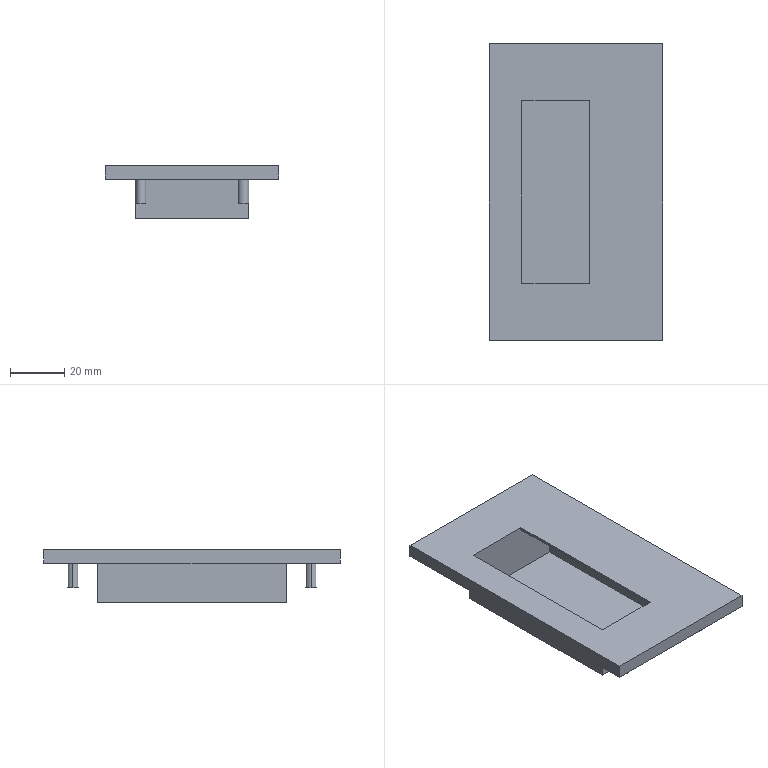Component | SolidWorks | SYM0671-81-200-1_SYMA1-51a_mis_uwuan109.5-b-1 | 1 solid | 30 faces | box 64 x 109.5 x 19.5 mm | volume 28880 mm3 | plane 22 | cylinder 8 | commonest cylinder face diameters 4 x8
build123d program:
from build123d import *

# Parameters (mm, degrees)
SKETCH_1_W           = 64
SKETCH_1_H           = 109.5
EXTRUDE1_DEPTH       = 5
SKETCH_6_W           = 42
SKETCH_6_H           = 69.5
EXTRUDE5_DEPTH       = 14.5
SKETCH1_W            = 25
SKETCH1_H            = 67.5
CUT_EXTRUDE1_DEPTH   = 18.5
SKETCH2_W            = 17.5
SKETCH2_H            = 67.5
CUT_EXTRUDE2_DEPTH   = 15
SKETCH3_R            = 2
EXTRUDE1_2_DEPTH     = 9
LPATTERN1_COUNT      = 2
LPATTERN1_PITCH      = 38
LPATTERN1_COUNT_DIR2 = 2
LPATTERN1_PITCH_DIR2 = 88


with BuildPart() as part:
    # Sketch 1 → Extrude1 (new body)
    with BuildSketch(Plane.XY):
        Rectangle(SKETCH_1_W, SKETCH_1_H)
    extrude(amount=EXTRUDE1_DEPTH)

    # Sketch 6 → Extrude5 (add)
    with BuildSketch(Plane.XY):
        Rectangle(SKETCH_6_W, SKETCH_6_H)
    extrude(amount=-EXTRUDE5_DEPTH)

    # Sketch1 → Cut-Extrude1 (cut)
    with BuildSketch(Plane.XY.offset(5)):
        with Locations((7.5, 0)):
            Rectangle(SKETCH1_W, SKETCH1_H)
    extrude(amount=-CUT_EXTRUDE1_DEPTH, mode=Mode.SUBTRACT)

    # Sketch2 → Cut-Extrude2 (cut)
    with BuildSketch(Plane(origin=(-5, 0, 0), x_dir=(0, 0, -1), z_dir=(1, 0, 0))):
        with Locations((4.75, 0)):
            Rectangle(SKETCH2_W, SKETCH2_H)
    extrude(amount=-CUT_EXTRUDE2_DEPTH, mode=Mode.SUBTRACT)

    # Sketch3 → Extrude1_2 (add)
    with BuildSketch(Plane(origin=(0, 0, 0), x_dir=(-1, 0, 0), z_dir=(0, 0, -1))):
        with Locations(Location((19, 44, 0), (0, 0, 180))):
            Circle(SKETCH3_R)
    extrude1_2 = extrude(amount=EXTRUDE1_2_DEPTH)

    # LPattern1: Extrude1_2 2 × 2
    with Locations(*[(i * LPATTERN1_PITCH, -j * LPATTERN1_PITCH_DIR2, 0) for i in range(LPATTERN1_COUNT) for j in range(LPATTERN1_COUNT_DIR2) if (i, j) != (0, 0)]):
        add(extrude1_2)


solid = part.part

# Placed as in the assembly
solid = solid.moved(Location((0.2513, -14.857, 1051.018), (0, 0, 180)))
STEP:
#1=CARTESIAN_POINT('',(-0.6594,1.147,41.024));
#2=VERTEX_POINT('',#1);
#3=CARTESIAN_POINT('',(-0.8169,1.147,41.024));
#4=VERTEX_POINT('',#3);
#5=CARTESIAN_POINT('',(-0.7381,1.147,41.024));
#6=DIRECTION('',(0.,0.,-1.));
#7=DIRECTION('',(1.,0.,0.));
#8=AXIS2_PLACEMENT_3D('',#5,#6,#7);
#9=CIRCLE('',#8,0.07874);
#10=EDGE_CURVE('',#2,#4,#9,.T.);
#11=ORIENTED_EDGE('',*,*,#10,.F.);
#12=CARTESIAN_POINT('',(-0.6594,1.147,41.379));
#13=VERTEX_POINT('',#12);
#14=CARTESIAN_POINT('',(-0.6594,1.147,41.024));
#15=DIRECTION('',(0.,0.,1.));
#16=VECTOR('',#15,39.37);
#17=LINE('',#14,#16);
#18=EDGE_CURVE('',#2,#13,#17,.T.);
#19=ORIENTED_EDGE('',*,*,#18,.T.);
#20=CARTESIAN_POINT('',(-0.8169,1.147,41.379));
#21=VERTEX_POINT('',#20);
#22=CARTESIAN_POINT('',(-0.7381,1.147,41.379));
#23=DIRECTION('',(0.,0.,-1.));
#24=DIRECTION('',(-1.,-0.,0.));
#25=AXIS2_PLACEMENT_3D('',#22,#23,#24);
#26=CIRCLE('',#25,0.07874);
#27=EDGE_CURVE('',#13,#21,#26,.T.);
#28=ORIENTED_EDGE('',*,*,#27,.T.);
#29=CARTESIAN_POINT('',(-0.8169,1.147,41.024));
#30=DIRECTION('',(0.,0.,1.));
#31=VECTOR('',#30,39.37);
#32=LINE('',#29,#31);
#33=EDGE_CURVE('',#4,#21,#32,.T.);
#34=ORIENTED_EDGE('',*,*,#33,.F.);
#35=EDGE_LOOP('',(#11,#19,#28,#34));
#36=FACE_OUTER_BOUND('',#35,.T.);
#37=CARTESIAN_POINT('',(-0.7381,1.147,41.024));
#38=DIRECTION('',(0.,0.,1.));
#39=DIRECTION('',(-1.,0.,0.));
#40=AXIS2_PLACEMENT_3D('',#37,#38,#39);
#41=CYLINDRICAL_SURFACE('',#40,0.07874);
#42=ADVANCED_FACE('',(#36),#41,.T.);
#43=CARTESIAN_POINT('',(0.8367,1.147,41.024));
#44=VERTEX_POINT('',#43);
#45=CARTESIAN_POINT('',(0.6792,1.147,41.024));
#46=VERTEX_POINT('',#45);
#47=CARTESIAN_POINT('',(0.7579,1.147,41.024));
#48=DIRECTION('',(0.,0.,-1.));
#49=DIRECTION('',(1.,0.,0.));
#50=AXIS2_PLACEMENT_3D('',#47,#48,#49);
#51=CIRCLE('',#50,0.07874);
#52=EDGE_CURVE('',#44,#46,#51,.T.);
#53=ORIENTED_EDGE('',*,*,#52,.F.);
#54=CARTESIAN_POINT('',(0.8367,1.147,41.379));
#55=VERTEX_POINT('',#54);
#56=CARTESIAN_POINT('',(0.8367,1.147,41.024));
#57=DIRECTION('',(0.,0.,1.));
#58=VECTOR('',#57,39.37);
#59=LINE('',#56,#58);
#60=EDGE_CURVE('',#44,#55,#59,.T.);
#61=ORIENTED_EDGE('',*,*,#60,.T.);
#62=CARTESIAN_POINT('',(0.6792,1.147,41.379));
#63=VERTEX_POINT('',#62);
#64=CARTESIAN_POINT('',(0.7579,1.147,41.379));
#65=DIRECTION('',(0.,0.,-1.));
#66=DIRECTION('',(-1.,-0.,0.));
#67=AXIS2_PLACEMENT_3D('',#64,#65,#66);
#68=CIRCLE('',#67,0.07874);
#69=EDGE_CURVE('',#55,#63,#68,.T.);
#70=ORIENTED_EDGE('',*,*,#69,.T.);
#71=CARTESIAN_POINT('',(0.6792,1.147,41.024));
#72=DIRECTION('',(0.,0.,1.));
#73=VECTOR('',#72,39.37);
#74=LINE('',#71,#73);
#75=EDGE_CURVE('',#46,#63,#74,.T.);
#76=ORIENTED_EDGE('',*,*,#75,.F.);
#77=EDGE_LOOP('',(#53,#61,#70,#76));
#78=FACE_OUTER_BOUND('',#77,.T.);
#79=CARTESIAN_POINT('',(0.7579,1.147,41.024));
#80=DIRECTION('',(0.,0.,1.));
#81=DIRECTION('',(-1.,0.,0.));
#82=AXIS2_PLACEMENT_3D('',#79,#80,#81);
#83=CYLINDRICAL_SURFACE('',#82,0.07874);
#84=ADVANCED_FACE('',(#78),#83,.T.);
#85=CARTESIAN_POINT('',(-0.6594,-2.317,41.024));
#86=VERTEX_POINT('',#85);
#87=CARTESIAN_POINT('',(-0.8169,-2.317,41.024));
#88=VERTEX_POINT('',#87);
#89=CARTESIAN_POINT('',(-0.7381,-2.317,41.024));
#90=DIRECTION('',(0.,0.,-1.));
#91=DIRECTION('',(1.,0.,0.));
#92=AXIS2_PLACEMENT_3D('',#89,#90,#91);
#93=CIRCLE('',#92,0.07874);
#94=EDGE_CURVE('',#86,#88,#93,.T.);
#95=ORIENTED_EDGE('',*,*,#94,.F.);
#96=CARTESIAN_POINT('',(-0.6594,-2.317,41.379));
#97=VERTEX_POINT('',#96);
#98=CARTESIAN_POINT('',(-0.6594,-2.317,41.024));
#99=DIRECTION('',(0.,0.,1.));
#100=VECTOR('',#99,39.37);
#101=LINE('',#98,#100);
#102=EDGE_CURVE('',#86,#97,#101,.T.);
#103=ORIENTED_EDGE('',*,*,#102,.T.);
#104=CARTESIAN_POINT('',(-0.8169,-2.317,41.379));
#105=VERTEX_POINT('',#104);
#106=CARTESIAN_POINT('',(-0.7381,-2.317,41.379));
#107=DIRECTION('',(0.,0.,-1.));
#108=DIRECTION('',(-1.,0.,0.));
#109=AXIS2_PLACEMENT_3D('',#106,#107,#108);
#110=CIRCLE('',#109,0.07874);
#111=EDGE_CURVE('',#97,#105,#110,.T.);
#112=ORIENTED_EDGE('',*,*,#111,.T.);
#113=CARTESIAN_POINT('',(-0.8169,-2.317,41.024));
#114=DIRECTION('',(0.,0.,1.));
#115=VECTOR('',#114,39.37);
#116=LINE('',#113,#115);
#117=EDGE_CURVE('',#88,#105,#116,.T.);
#118=ORIENTED_EDGE('',*,*,#117,.F.);
#119=EDGE_LOOP('',(#95,#103,#112,#118));
#120=FACE_OUTER_BOUND('',#119,.T.);
#121=CARTESIAN_POINT('',(-0.7381,-2.317,41.024));
#122=DIRECTION('',(0.,0.,1.));
#123=DIRECTION('',(-1.,0.,0.));
#124=AXIS2_PLACEMENT_3D('',#121,#122,#123);
#125=CYLINDRICAL_SURFACE('',#124,0.07874);
#126=ADVANCED_FACE('',(#120),#125,.T.);
#127=CARTESIAN_POINT('',(0.8367,-2.317,41.024));
#128=VERTEX_POINT('',#127);
#129=CARTESIAN_POINT('',(0.6792,-2.317,41.024));
#130=VERTEX_POINT('',#129);
#131=CARTESIAN_POINT('',(0.7579,-2.317,41.024));
#132=DIRECTION('',(0.,0.,-1.));
#133=DIRECTION('',(1.,0.,0.));
#134=AXIS2_PLACEMENT_3D('',#131,#132,#133);
#135=CIRCLE('',#134,0.07874);
#136=EDGE_CURVE('',#128,#130,#135,.T.);
#137=ORIENTED_EDGE('',*,*,#136,.F.);
#138=CARTESIAN_POINT('',(0.8367,-2.317,41.379));
#139=VERTEX_POINT('',#138);
#140=CARTESIAN_POINT('',(0.8367,-2.317,41.024));
#141=DIRECTION('',(0.,0.,1.));
#142=VECTOR('',#141,39.37);
#143=LINE('',#140,#142);
#144=EDGE_CURVE('',#128,#139,#143,.T.);
#145=ORIENTED_EDGE('',*,*,#144,.T.);
#146=CARTESIAN_POINT('',(0.6792,-2.317,41.379));
#147=VERTEX_POINT('',#146);
#148=CARTESIAN_POINT('',(0.7579,-2.317,41.379));
#149=DIRECTION('',(0.,0.,-1.));
#150=DIRECTION('',(-1.,0.,0.));
#151=AXIS2_PLACEMENT_3D('',#148,#149,#150);
#152=CIRCLE('',#151,0.07874);
#153=EDGE_CURVE('',#139,#147,#152,.T.);
#154=ORIENTED_EDGE('',*,*,#153,.T.);
#155=CARTESIAN_POINT('',(0.6792,-2.317,41.024));
#156=DIRECTION('',(0.,0.,1.));
#157=VECTOR('',#156,39.37);
#158=LINE('',#155,#157);
#159=EDGE_CURVE('',#130,#147,#158,.T.);
#160=ORIENTED_EDGE('',*,*,#159,.F.);
#161=EDGE_LOOP('',(#137,#145,#154,#160));
#162=FACE_OUTER_BOUND('',#161,.T.);
#163=CARTESIAN_POINT('',(0.7579,-2.317,41.024));
#164=DIRECTION('',(0.,0.,1.));
#165=DIRECTION('',(-1.,0.,0.));
#166=AXIS2_PLACEMENT_3D('',#163,#164,#165);
#167=CYLINDRICAL_SURFACE('',#166,0.07874);
#168=ADVANCED_FACE('',(#162),#167,.T.);
#169=CARTESIAN_POINT('',(0.7579,-2.317,41.379));
#170=DIRECTION('',(0.,0.,-1.));
#171=DIRECTION('',(-1.,0.,0.));
#172=AXIS2_PLACEMENT_3D('',#169,#170,#171);
#173=CIRCLE('',#172,0.07874);
#174=EDGE_CURVE('',#147,#139,#173,.T.);
#175=ORIENTED_EDGE('',*,*,#174,.F.);
#176=ORIENTED_EDGE('',*,*,#153,.F.);
#177=EDGE_LOOP('',(#175,#176));
#178=FACE_BOUND('',#177,.T.);
#179=CARTESIAN_POINT('',(0.8367,0.7832,41.379));
#180=VERTEX_POINT('',#179);
#181=CARTESIAN_POINT('',(-0.8169,0.7832,41.379));
#182=VERTEX_POINT('',#181);
#183=CARTESIAN_POINT('',(-0.8169,0.7832,41.379));
#184=DIRECTION('',(-1.,-0.,0.));
#185=VECTOR('',#184,39.37);
#186=LINE('',#183,#185);
#187=EDGE_CURVE('',#180,#182,#186,.T.);
#188=ORIENTED_EDGE('',*,*,#187,.T.);
#189=CARTESIAN_POINT('',(-0.8169,-1.953,41.379));
#190=VERTEX_POINT('',#189);
#191=CARTESIAN_POINT('',(-0.8169,-1.953,41.379));
#192=DIRECTION('',(0.,-1.,0.));
#193=VECTOR('',#192,39.37);
#194=LINE('',#191,#193);
#195=EDGE_CURVE('',#182,#190,#194,.T.);
#196=ORIENTED_EDGE('',*,*,#195,.T.);
#197=CARTESIAN_POINT('',(0.8367,-1.953,41.379));
#198=VERTEX_POINT('',#197);
#199=CARTESIAN_POINT('',(-0.8169,-1.953,41.379));
#200=DIRECTION('',(1.,0.,0.));
#201=VECTOR('',#200,39.37);
#202=LINE('',#199,#201);
#203=EDGE_CURVE('',#190,#198,#202,.T.);
#204=ORIENTED_EDGE('',*,*,#203,.T.);
#205=CARTESIAN_POINT('',(0.8367,-1.953,41.379));
#206=DIRECTION('',(-0.,1.,0.));
#207=VECTOR('',#206,39.37);
#208=LINE('',#205,#207);
#209=EDGE_CURVE('',#198,#180,#208,.T.);
#210=ORIENTED_EDGE('',*,*,#209,.T.);
#211=EDGE_LOOP('',(#188,#196,#204,#210));
#212=FACE_BOUND('',#211,.T.);
#213=CARTESIAN_POINT('',(1.27,-2.74,41.379));
#214=VERTEX_POINT('',#213);
#215=CARTESIAN_POINT('',(1.27,1.571,41.379));
#216=VERTEX_POINT('',#215);
#217=CARTESIAN_POINT('',(1.27,-2.74,41.379));
#218=DIRECTION('',(-0.,1.,0.));
#219=VECTOR('',#218,39.37);
#220=LINE('',#217,#219);
#221=EDGE_CURVE('',#214,#216,#220,.T.);
#222=ORIENTED_EDGE('',*,*,#221,.F.);
#223=CARTESIAN_POINT('',(-1.25,-2.74,41.379));
#224=VERTEX_POINT('',#223);
#225=CARTESIAN_POINT('',(1.27,-2.74,41.379));
#226=DIRECTION('',(1.,0.,0.));
#227=VECTOR('',#226,39.37);
#228=LINE('',#225,#227);
#229=EDGE_CURVE('',#224,#214,#228,.T.);
#230=ORIENTED_EDGE('',*,*,#229,.F.);
#231=CARTESIAN_POINT('',(-1.25,1.571,41.379));
#232=VERTEX_POINT('',#231);
#233=CARTESIAN_POINT('',(-1.25,-2.74,41.379));
#234=DIRECTION('',(0.,-1.,0.));
#235=VECTOR('',#234,39.37);
#236=LINE('',#233,#235);
#237=EDGE_CURVE('',#232,#224,#236,.T.);
#238=ORIENTED_EDGE('',*,*,#237,.F.);
#239=CARTESIAN_POINT('',(1.27,1.571,41.379));
#240=DIRECTION('',(-1.,-0.,0.));
#241=VECTOR('',#240,39.37);
#242=LINE('',#239,#241);
#243=EDGE_CURVE('',#216,#232,#242,.T.);
#244=ORIENTED_EDGE('',*,*,#243,.F.);
#245=EDGE_LOOP('',(#222,#230,#238,#244));
#246=FACE_OUTER_BOUND('',#245,.T.);
#247=CARTESIAN_POINT('',(-0.7381,-2.317,41.379));
#248=DIRECTION('',(0.,0.,-1.));
#249=DIRECTION('',(-1.,0.,0.));
#250=AXIS2_PLACEMENT_3D('',#247,#248,#249);
#251=CIRCLE('',#250,0.07874);
#252=EDGE_CURVE('',#105,#97,#251,.T.);
#253=ORIENTED_EDGE('',*,*,#252,.F.);
#254=ORIENTED_EDGE('',*,*,#111,.F.);
#255=EDGE_LOOP('',(#253,#254));
#256=FACE_BOUND('',#255,.T.);
#257=CARTESIAN_POINT('',(0.7579,1.147,41.379));
#258=DIRECTION('',(0.,0.,-1.));
#259=DIRECTION('',(-1.,0.,0.));
#260=AXIS2_PLACEMENT_3D('',#257,#258,#259);
#261=CIRCLE('',#260,0.07874);
#262=EDGE_CURVE('',#63,#55,#261,.T.);
#263=ORIENTED_EDGE('',*,*,#262,.F.);
#264=ORIENTED_EDGE('',*,*,#69,.F.);
#265=EDGE_LOOP('',(#263,#264));
#266=FACE_BOUND('',#265,.T.);
#267=CARTESIAN_POINT('',(-0.7381,1.147,41.379));
#268=DIRECTION('',(0.,0.,-1.));
#269=DIRECTION('',(-1.,0.,0.));
#270=AXIS2_PLACEMENT_3D('',#267,#268,#269);
#271=CIRCLE('',#270,0.07874);
#272=EDGE_CURVE('',#21,#13,#271,.T.);
#273=ORIENTED_EDGE('',*,*,#272,.F.);
#274=ORIENTED_EDGE('',*,*,#27,.F.);
#275=EDGE_LOOP('',(#273,#274));
#276=FACE_BOUND('',#275,.T.);
#277=CARTESIAN_POINT('',(1.27,1.571,41.379));
#278=DIRECTION('',(0.,0.,1.));
#279=DIRECTION('',(-1.,-0.,0.));
#280=AXIS2_PLACEMENT_3D('',#277,#278,#279);
#281=PLANE('',#280);
#282=ADVANCED_FACE('',(#178,#212,#246,#256,#266,#276),#281,.F.);
#283=ORIENTED_EDGE('',*,*,#221,.T.);
#284=CARTESIAN_POINT('',(1.27,1.571,41.575));
#285=VERTEX_POINT('',#284);
#286=CARTESIAN_POINT('',(1.27,1.571,41.575));
#287=DIRECTION('',(0.,0.,-1.));
#288=VECTOR('',#287,39.37);
#289=LINE('',#286,#288);
#290=EDGE_CURVE('',#285,#216,#289,.T.);
#291=ORIENTED_EDGE('',*,*,#290,.F.);
#292=CARTESIAN_POINT('',(1.27,-2.74,41.575));
#293=VERTEX_POINT('',#292);
#294=CARTESIAN_POINT('',(1.27,-2.74,41.575));
#295=DIRECTION('',(-0.,1.,0.));
#296=VECTOR('',#295,39.37);
#297=LINE('',#294,#296);
#298=EDGE_CURVE('',#293,#285,#297,.T.);
#299=ORIENTED_EDGE('',*,*,#298,.F.);
#300=CARTESIAN_POINT('',(1.27,-2.74,41.575));
#301=DIRECTION('',(0.,0.,-1.));
#302=VECTOR('',#301,39.37);
#303=LINE('',#300,#302);
#304=EDGE_CURVE('',#293,#214,#303,.T.);
#305=ORIENTED_EDGE('',*,*,#304,.T.);
#306=EDGE_LOOP('',(#283,#291,#299,#305));
#307=FACE_OUTER_BOUND('',#306,.T.);
#308=CARTESIAN_POINT('',(1.27,-2.74,41.575));
#309=DIRECTION('',(-1.,-0.,0.));
#310=DIRECTION('',(0.,-1.,0.));
#311=AXIS2_PLACEMENT_3D('',#308,#309,#310);
#312=PLANE('',#311);
#313=ADVANCED_FACE('',(#307),#312,.F.);
#314=ORIENTED_EDGE('',*,*,#243,.T.);
#315=CARTESIAN_POINT('',(-1.25,1.571,41.575));
#316=VERTEX_POINT('',#315);
#317=CARTESIAN_POINT('',(-1.25,1.571,41.575));
#318=DIRECTION('',(0.,0.,-1.));
#319=VECTOR('',#318,39.37);
#320=LINE('',#317,#319);
#321=EDGE_CURVE('',#316,#232,#320,.T.);
#322=ORIENTED_EDGE('',*,*,#321,.F.);
#323=CARTESIAN_POINT('',(1.27,1.571,41.575));
#324=DIRECTION('',(-1.,-0.,0.));
#325=VECTOR('',#324,39.37);
#326=LINE('',#323,#325);
#327=EDGE_CURVE('',#285,#316,#326,.T.);
#328=ORIENTED_EDGE('',*,*,#327,.F.);
#329=ORIENTED_EDGE('',*,*,#290,.T.);
#330=EDGE_LOOP('',(#314,#322,#328,#329));
#331=FACE_OUTER_BOUND('',#330,.T.);
#332=CARTESIAN_POINT('',(1.27,1.571,41.575));
#333=DIRECTION('',(0.,-1.,0.));
#334=DIRECTION('',(1.,0.,0.));
#335=AXIS2_PLACEMENT_3D('',#332,#333,#334);
#336=PLANE('',#335);
#337=ADVANCED_FACE('',(#331),#336,.F.);
#338=ORIENTED_EDGE('',*,*,#237,.T.);
#339=CARTESIAN_POINT('',(-1.25,-2.74,41.575));
#340=VERTEX_POINT('',#339);
#341=CARTESIAN_POINT('',(-1.25,-2.74,41.575));
#342=DIRECTION('',(0.,0.,-1.));
#343=VECTOR('',#342,39.37);
#344=LINE('',#341,#343);
#345=EDGE_CURVE('',#340,#224,#344,.T.);
#346=ORIENTED_EDGE('',*,*,#345,.F.);
#347=CARTESIAN_POINT('',(-1.25,-2.74,41.575));
#348=DIRECTION('',(0.,-1.,0.));
#349=VECTOR('',#348,39.37);
#350=LINE('',#347,#349);
#351=EDGE_CURVE('',#316,#340,#350,.T.);
#352=ORIENTED_EDGE('',*,*,#351,.F.);
#353=ORIENTED_EDGE('',*,*,#321,.T.);
#354=EDGE_LOOP('',(#338,#346,#352,#353));
#355=FACE_OUTER_BOUND('',#354,.T.);
#356=CARTESIAN_POINT('',(-1.25,-2.74,41.575));
#357=DIRECTION('',(1.,0.,0.));
#358=DIRECTION('',(-0.,1.,0.));
#359=AXIS2_PLACEMENT_3D('',#356,#357,#358);
#360=PLANE('',#359);
#361=ADVANCED_FACE('',(#355),#360,.F.);
#362=ORIENTED_EDGE('',*,*,#229,.T.);
#363=ORIENTED_EDGE('',*,*,#304,.F.);
#364=CARTESIAN_POINT('',(1.27,-2.74,41.575));
#365=DIRECTION('',(1.,0.,0.));
#366=VECTOR('',#365,39.37);
#367=LINE('',#364,#366);
#368=EDGE_CURVE('',#340,#293,#367,.T.);
#369=ORIENTED_EDGE('',*,*,#368,.F.);
#370=ORIENTED_EDGE('',*,*,#345,.T.);
#371=EDGE_LOOP('',(#362,#363,#369,#370));
#372=FACE_OUTER_BOUND('',#371,.T.);
#373=CARTESIAN_POINT('',(1.27,-2.74,41.575));
#374=DIRECTION('',(-0.,1.,0.));
#375=DIRECTION('',(-1.,-0.,0.));
#376=AXIS2_PLACEMENT_3D('',#373,#374,#375);
#377=PLANE('',#376);
#378=ADVANCED_FACE('',(#372),#377,.F.);
#379=CARTESIAN_POINT('',(0.2067,0.7438,41.575));
#380=VERTEX_POINT('',#379);
#381=CARTESIAN_POINT('',(-0.7775,0.7438,41.575));
#382=VERTEX_POINT('',#381);
#383=CARTESIAN_POINT('',(0.2067,0.7438,41.575));
#384=DIRECTION('',(-1.,-0.,0.));
#385=VECTOR('',#384,39.37);
#386=LINE('',#383,#385);
#387=EDGE_CURVE('',#380,#382,#386,.T.);
#388=ORIENTED_EDGE('',*,*,#387,.F.);
#389=CARTESIAN_POINT('',(0.2067,-1.914,41.575));
#390=VERTEX_POINT('',#389);
#391=CARTESIAN_POINT('',(0.2067,-1.914,41.575));
#392=DIRECTION('',(-0.,1.,0.));
#393=VECTOR('',#392,39.37);
#394=LINE('',#391,#393);
#395=EDGE_CURVE('',#390,#380,#394,.T.);
#396=ORIENTED_EDGE('',*,*,#395,.F.);
#397=CARTESIAN_POINT('',(-0.7775,-1.914,41.575));
#398=VERTEX_POINT('',#397);
#399=CARTESIAN_POINT('',(-0.7775,-1.914,41.575));
#400=DIRECTION('',(1.,0.,0.));
#401=VECTOR('',#400,39.37);
#402=LINE('',#399,#401);
#403=EDGE_CURVE('',#398,#390,#402,.T.);
#404=ORIENTED_EDGE('',*,*,#403,.F.);
#405=CARTESIAN_POINT('',(-0.7775,0.7438,41.575));
#406=DIRECTION('',(0.,-1.,0.));
#407=VECTOR('',#406,39.37);
#408=LINE('',#405,#407);
#409=EDGE_CURVE('',#382,#398,#408,.T.);
#410=ORIENTED_EDGE('',*,*,#409,.F.);
#411=EDGE_LOOP('',(#388,#396,#404,#410));
#412=FACE_BOUND('',#411,.T.);
#413=ORIENTED_EDGE('',*,*,#298,.T.);
#414=ORIENTED_EDGE('',*,*,#327,.T.);
#415=ORIENTED_EDGE('',*,*,#351,.T.);
#416=ORIENTED_EDGE('',*,*,#368,.T.);
#417=EDGE_LOOP('',(#413,#414,#415,#416));
#418=FACE_OUTER_BOUND('',#417,.T.);
#419=CARTESIAN_POINT('',(1.27,1.571,41.575));
#420=DIRECTION('',(0.,0.,1.));
#421=DIRECTION('',(-1.,-0.,0.));
#422=AXIS2_PLACEMENT_3D('',#419,#420,#421);
#423=PLANE('',#422);
#424=ADVANCED_FACE('',(#412,#418),#423,.T.);
#425=ORIENTED_EDGE('',*,*,#195,.F.);
#426=CARTESIAN_POINT('',(-0.8169,0.7832,40.808));
#427=VERTEX_POINT('',#426);
#428=CARTESIAN_POINT('',(-0.8169,0.7832,40.808));
#429=DIRECTION('',(0.,0.,1.));
#430=VECTOR('',#429,39.37);
#431=LINE('',#428,#430);
#432=EDGE_CURVE('',#427,#182,#431,.T.);
#433=ORIENTED_EDGE('',*,*,#432,.F.);
#434=CARTESIAN_POINT('',(-0.8169,-1.953,40.808));
#435=VERTEX_POINT('',#434);
#436=CARTESIAN_POINT('',(-0.8169,-1.953,40.808));
#437=DIRECTION('',(0.,-1.,0.));
#438=VECTOR('',#437,39.37);
#439=LINE('',#436,#438);
#440=EDGE_CURVE('',#427,#435,#439,.T.);
#441=ORIENTED_EDGE('',*,*,#440,.T.);
#442=CARTESIAN_POINT('',(-0.8169,-1.953,40.808));
#443=DIRECTION('',(0.,0.,1.));
#444=VECTOR('',#443,39.37);
#445=LINE('',#442,#444);
#446=EDGE_CURVE('',#435,#190,#445,.T.);
#447=ORIENTED_EDGE('',*,*,#446,.T.);
#448=EDGE_LOOP('',(#425,#433,#441,#447));
#449=FACE_OUTER_BOUND('',#448,.T.);
#450=CARTESIAN_POINT('',(-0.8169,-1.953,40.808));
#451=DIRECTION('',(-1.,-0.,0.));
#452=DIRECTION('',(0.,-1.,0.));
#453=AXIS2_PLACEMENT_3D('',#450,#451,#452);
#454=PLANE('',#453);
#455=ADVANCED_FACE('',(#449),#454,.T.);
#456=ORIENTED_EDGE('',*,*,#187,.F.);
#457=CARTESIAN_POINT('',(0.8367,0.7832,40.808));
#458=VERTEX_POINT('',#457);
#459=CARTESIAN_POINT('',(0.8367,0.7832,40.808));
#460=DIRECTION('',(0.,0.,1.));
#461=VECTOR('',#460,39.37);
#462=LINE('',#459,#461);
#463=EDGE_CURVE('',#458,#180,#462,.T.);
#464=ORIENTED_EDGE('',*,*,#463,.F.);
#465=CARTESIAN_POINT('',(-0.8169,0.7832,40.808));
#466=DIRECTION('',(-1.,-0.,0.));
#467=VECTOR('',#466,39.37);
#468=LINE('',#465,#467);
#469=EDGE_CURVE('',#458,#427,#468,.T.);
#470=ORIENTED_EDGE('',*,*,#469,.T.);
#471=ORIENTED_EDGE('',*,*,#432,.T.);
#472=EDGE_LOOP('',(#456,#464,#470,#471));
#473=FACE_OUTER_BOUND('',#472,.T.);
#474=CARTESIAN_POINT('',(-0.8169,0.7832,40.808));
#475=DIRECTION('',(-0.,1.,0.));
#476=DIRECTION('',(-1.,-0.,0.));
#477=AXIS2_PLACEMENT_3D('',#474,#475,#476);
#478=PLANE('',#477);
#479=ADVANCED_FACE('',(#473),#478,.T.);
#480=ORIENTED_EDGE('',*,*,#209,.F.);
#481=CARTESIAN_POINT('',(0.8367,-1.953,40.808));
#482=VERTEX_POINT('',#481);
#483=CARTESIAN_POINT('',(0.8367,-1.953,40.808));
#484=DIRECTION('',(0.,0.,1.));
#485=VECTOR('',#484,39.37);
#486=LINE('',#483,#485);
#487=EDGE_CURVE('',#482,#198,#486,.T.);
#488=ORIENTED_EDGE('',*,*,#487,.F.);
#489=CARTESIAN_POINT('',(0.8367,-1.953,40.808));
#490=DIRECTION('',(-0.,1.,0.));
#491=VECTOR('',#490,39.37);
#492=LINE('',#489,#491);
#493=EDGE_CURVE('',#482,#458,#492,.T.);
#494=ORIENTED_EDGE('',*,*,#493,.T.);
#495=ORIENTED_EDGE('',*,*,#463,.T.);
#496=EDGE_LOOP('',(#480,#488,#494,#495));
#497=FACE_OUTER_BOUND('',#496,.T.);
#498=CARTESIAN_POINT('',(0.8367,-1.953,40.808));
#499=DIRECTION('',(1.,0.,0.));
#500=DIRECTION('',(-0.,1.,0.));
#501=AXIS2_PLACEMENT_3D('',#498,#499,#500);
#502=PLANE('',#501);
#503=ADVANCED_FACE('',(#497),#502,.T.);
#504=ORIENTED_EDGE('',*,*,#203,.F.);
#505=ORIENTED_EDGE('',*,*,#446,.F.);
#506=CARTESIAN_POINT('',(-0.8169,-1.953,40.808));
#507=DIRECTION('',(1.,0.,0.));
#508=VECTOR('',#507,39.37);
#509=LINE('',#506,#508);
#510=EDGE_CURVE('',#435,#482,#509,.T.);
#511=ORIENTED_EDGE('',*,*,#510,.T.);
#512=ORIENTED_EDGE('',*,*,#487,.T.);
#513=EDGE_LOOP('',(#504,#505,#511,#512));
#514=FACE_OUTER_BOUND('',#513,.T.);
#515=CARTESIAN_POINT('',(-0.8169,-1.953,40.808));
#516=DIRECTION('',(0.,-1.,0.));
#517=DIRECTION('',(1.,0.,0.));
#518=AXIS2_PLACEMENT_3D('',#515,#516,#517);
#519=PLANE('',#518);
#520=ADVANCED_FACE('',(#514),#519,.T.);
#521=ORIENTED_EDGE('',*,*,#440,.F.);
#522=ORIENTED_EDGE('',*,*,#469,.F.);
#523=ORIENTED_EDGE('',*,*,#493,.F.);
#524=ORIENTED_EDGE('',*,*,#510,.F.);
#525=EDGE_LOOP('',(#521,#522,#523,#524));
#526=FACE_OUTER_BOUND('',#525,.T.);
#527=CARTESIAN_POINT('',(-0.8169,0.7832,40.808));
#528=DIRECTION('',(0.,0.,-1.));
#529=DIRECTION('',(1.,0.,0.));
#530=AXIS2_PLACEMENT_3D('',#527,#528,#529);
#531=PLANE('',#530);
#532=ADVANCED_FACE('',(#526),#531,.T.);
#533=ORIENTED_EDGE('',*,*,#387,.T.);
#534=CARTESIAN_POINT('',(-0.7775,0.7438,40.847));
#535=VERTEX_POINT('',#534);
#536=CARTESIAN_POINT('',(-0.7775,0.7438,40.847));
#537=DIRECTION('',(0.,0.,1.));
#538=VECTOR('',#537,39.37);
#539=LINE('',#536,#538);
#540=EDGE_CURVE('',#535,#382,#539,.T.);
#541=ORIENTED_EDGE('',*,*,#540,.F.);
#542=CARTESIAN_POINT('',(0.7973,0.7438,40.847));
#543=VERTEX_POINT('',#542);
#544=CARTESIAN_POINT('',(0.2067,0.7438,40.847));
#545=DIRECTION('',(-1.,-0.,0.));
#546=VECTOR('',#545,39.37);
#547=LINE('',#544,#546);
#548=EDGE_CURVE('',#543,#535,#547,.T.);
#549=ORIENTED_EDGE('',*,*,#548,.F.);
#550=CARTESIAN_POINT('',(0.7973,0.7438,41.536));
#551=VERTEX_POINT('',#550);
#552=CARTESIAN_POINT('',(0.7973,0.7438,40.847));
#553=DIRECTION('',(0.,0.,-1.));
#554=VECTOR('',#553,39.37);
#555=LINE('',#552,#554);
#556=EDGE_CURVE('',#551,#543,#555,.T.);
#557=ORIENTED_EDGE('',*,*,#556,.F.);
#558=CARTESIAN_POINT('',(0.2067,0.7438,41.536));
#559=VERTEX_POINT('',#558);
#560=CARTESIAN_POINT('',(3.582,0.7438,41.536));
#561=DIRECTION('',(-1.,-0.,0.));
#562=VECTOR('',#561,39.37);
#563=LINE('',#560,#562);
#564=EDGE_CURVE('',#551,#559,#563,.T.);
#565=ORIENTED_EDGE('',*,*,#564,.T.);
#566=CARTESIAN_POINT('',(0.2067,0.7438,40.847));
#567=DIRECTION('',(0.,0.,1.));
#568=VECTOR('',#567,39.37);
#569=LINE('',#566,#568);
#570=EDGE_CURVE('',#559,#380,#569,.T.);
#571=ORIENTED_EDGE('',*,*,#570,.T.);
#572=EDGE_LOOP('',(#533,#541,#549,#557,#565,#571));
#573=FACE_OUTER_BOUND('',#572,.T.);
#574=CARTESIAN_POINT('',(0.2067,0.7438,40.847));
#575=DIRECTION('',(-0.,1.,0.));
#576=DIRECTION('',(0.,0.,-1.));
#577=AXIS2_PLACEMENT_3D('',#574,#575,#576);
#578=PLANE('',#577);
#579=ADVANCED_FACE('',(#573),#578,.F.);
#580=ORIENTED_EDGE('',*,*,#570,.F.);
#581=CARTESIAN_POINT('',(0.2067,-1.914,41.536));
#582=VERTEX_POINT('',#581);
#583=CARTESIAN_POINT('',(0.2067,0.7438,41.536));
#584=DIRECTION('',(-0.,1.,0.));
#585=VECTOR('',#584,39.37);
#586=LINE('',#583,#585);
#587=EDGE_CURVE('',#582,#559,#586,.T.);
#588=ORIENTED_EDGE('',*,*,#587,.F.);
#589=CARTESIAN_POINT('',(0.2067,-1.914,40.847));
#590=DIRECTION('',(0.,0.,1.));
#591=VECTOR('',#590,39.37);
#592=LINE('',#589,#591);
#593=EDGE_CURVE('',#582,#390,#592,.T.);
#594=ORIENTED_EDGE('',*,*,#593,.T.);
#595=ORIENTED_EDGE('',*,*,#395,.T.);
#596=EDGE_LOOP('',(#580,#588,#594,#595));
#597=FACE_OUTER_BOUND('',#596,.T.);
#598=CARTESIAN_POINT('',(0.2067,-1.914,40.847));
#599=DIRECTION('',(1.,0.,0.));
#600=DIRECTION('',(-0.,1.,0.));
#601=AXIS2_PLACEMENT_3D('',#598,#599,#600);
#602=PLANE('',#601);
#603=ADVANCED_FACE('',(#597),#602,.F.);
#604=ORIENTED_EDGE('',*,*,#403,.T.);
#605=ORIENTED_EDGE('',*,*,#593,.F.);
#606=CARTESIAN_POINT('',(0.7973,-1.914,41.536));
#607=VERTEX_POINT('',#606);
#608=CARTESIAN_POINT('',(3.582,-1.914,41.536));
#609=DIRECTION('',(-1.,-0.,0.));
#610=VECTOR('',#609,39.37);
#611=LINE('',#608,#610);
#612=EDGE_CURVE('',#607,#582,#611,.T.);
#613=ORIENTED_EDGE('',*,*,#612,.F.);
#614=CARTESIAN_POINT('',(0.7973,-1.914,40.847));
#615=VERTEX_POINT('',#614);
#616=CARTESIAN_POINT('',(0.7973,-1.914,40.847));
#617=DIRECTION('',(0.,0.,1.));
#618=VECTOR('',#617,39.37);
#619=LINE('',#616,#618);
#620=EDGE_CURVE('',#615,#607,#619,.T.);
#621=ORIENTED_EDGE('',*,*,#620,.F.);
#622=CARTESIAN_POINT('',(-0.7775,-1.914,40.847));
#623=VERTEX_POINT('',#622);
#624=CARTESIAN_POINT('',(-0.7775,-1.914,40.847));
#625=DIRECTION('',(1.,0.,0.));
#626=VECTOR('',#625,39.37);
#627=LINE('',#624,#626);
#628=EDGE_CURVE('',#623,#615,#627,.T.);
#629=ORIENTED_EDGE('',*,*,#628,.F.);
#630=CARTESIAN_POINT('',(-0.7775,-1.914,40.847));
#631=DIRECTION('',(0.,0.,1.));
#632=VECTOR('',#631,39.37);
#633=LINE('',#630,#632);
#634=EDGE_CURVE('',#623,#398,#633,.T.);
#635=ORIENTED_EDGE('',*,*,#634,.T.);
#636=EDGE_LOOP('',(#604,#605,#613,#621,#629,#635));
#637=FACE_OUTER_BOUND('',#636,.T.);
#638=CARTESIAN_POINT('',(-0.7775,-1.914,40.847));
#639=DIRECTION('',(0.,-1.,0.));
#640=DIRECTION('',(1.,0.,0.));
#641=AXIS2_PLACEMENT_3D('',#638,#639,#640);
#642=PLANE('',#641);
#643=ADVANCED_FACE('',(#637),#642,.F.);
#644=ORIENTED_EDGE('',*,*,#409,.T.);
#645=ORIENTED_EDGE('',*,*,#634,.F.);
#646=CARTESIAN_POINT('',(-0.7775,0.7438,40.847));
#647=DIRECTION('',(0.,-1.,0.));
#648=VECTOR('',#647,39.37);
#649=LINE('',#646,#648);
#650=EDGE_CURVE('',#535,#623,#649,.T.);
#651=ORIENTED_EDGE('',*,*,#650,.F.);
#652=ORIENTED_EDGE('',*,*,#540,.T.);
#653=EDGE_LOOP('',(#644,#645,#651,#652));
#654=FACE_OUTER_BOUND('',#653,.T.);
#655=CARTESIAN_POINT('',(-0.7775,0.7438,40.847));
#656=DIRECTION('',(-1.,-0.,0.));
#657=DIRECTION('',(0.,-1.,0.));
#658=AXIS2_PLACEMENT_3D('',#655,#656,#657);
#659=PLANE('',#658);
#660=ADVANCED_FACE('',(#654),#659,.F.);
#661=ORIENTED_EDGE('',*,*,#548,.T.);
#662=ORIENTED_EDGE('',*,*,#650,.T.);
#663=ORIENTED_EDGE('',*,*,#628,.T.);
#664=CARTESIAN_POINT('',(0.7973,0.7438,40.847));
#665=DIRECTION('',(0.,-1.,0.));
#666=VECTOR('',#665,39.37);
#667=LINE('',#664,#666);
#668=EDGE_CURVE('',#543,#615,#667,.T.);
#669=ORIENTED_EDGE('',*,*,#668,.F.);
#670=EDGE_LOOP('',(#661,#662,#663,#669));
#671=FACE_OUTER_BOUND('',#670,.T.);
#672=CARTESIAN_POINT('',(-0.7775,0.7438,40.847));
#673=DIRECTION('',(0.,0.,1.));
#674=DIRECTION('',(-1.,-0.,0.));
#675=AXIS2_PLACEMENT_3D('',#672,#673,#674);
#676=PLANE('',#675);
#677=ADVANCED_FACE('',(#671),#676,.T.);
#678=ORIENTED_EDGE('',*,*,#668,.T.);
#679=ORIENTED_EDGE('',*,*,#620,.T.);
#680=CARTESIAN_POINT('',(0.7973,0.7438,41.536));
#681=DIRECTION('',(-0.,1.,0.));
#682=VECTOR('',#681,39.37);
#683=LINE('',#680,#682);
#684=EDGE_CURVE('',#607,#551,#683,.T.);
#685=ORIENTED_EDGE('',*,*,#684,.T.);
#686=ORIENTED_EDGE('',*,*,#556,.T.);
#687=EDGE_LOOP('',(#678,#679,#685,#686));
#688=FACE_OUTER_BOUND('',#687,.T.);
#689=CARTESIAN_POINT('',(0.7973,-1.953,40.808));
#690=DIRECTION('',(1.,0.,0.));
#691=DIRECTION('',(-0.,1.,0.));
#692=AXIS2_PLACEMENT_3D('',#689,#690,#691);
#693=PLANE('',#692);
#694=ADVANCED_FACE('',(#688),#693,.F.);
#695=ORIENTED_EDGE('',*,*,#612,.T.);
#696=ORIENTED_EDGE('',*,*,#587,.T.);
#697=ORIENTED_EDGE('',*,*,#564,.F.);
#698=ORIENTED_EDGE('',*,*,#684,.F.);
#699=EDGE_LOOP('',(#695,#696,#697,#698));
#700=FACE_OUTER_BOUND('',#699,.T.);
#701=CARTESIAN_POINT('',(3.582,0.7438,41.536));
#702=DIRECTION('',(0.,0.,1.));
#703=DIRECTION('',(-1.,-0.,0.));
#704=AXIS2_PLACEMENT_3D('',#701,#702,#703);
#705=PLANE('',#704);
#706=ADVANCED_FACE('',(#700),#705,.F.);
#707=ORIENTED_EDGE('',*,*,#144,.F.);
#708=CARTESIAN_POINT('',(0.7579,-2.317,41.024));
#709=DIRECTION('',(0.,0.,-1.));
#710=DIRECTION('',(1.,0.,0.));
#711=AXIS2_PLACEMENT_3D('',#708,#709,#710);
#712=CIRCLE('',#711,0.07874);
#713=EDGE_CURVE('',#130,#128,#712,.T.);
#714=ORIENTED_EDGE('',*,*,#713,.F.);
#715=ORIENTED_EDGE('',*,*,#159,.T.);
#716=ORIENTED_EDGE('',*,*,#174,.T.);
#717=EDGE_LOOP('',(#707,#714,#715,#716));
#718=FACE_OUTER_BOUND('',#717,.T.);
#719=CARTESIAN_POINT('',(0.7579,-2.317,41.024));
#720=DIRECTION('',(0.,0.,1.));
#721=DIRECTION('',(-1.,0.,0.));
#722=AXIS2_PLACEMENT_3D('',#719,#720,#721);
#723=CYLINDRICAL_SURFACE('',#722,0.07874);
#724=ADVANCED_FACE('',(#718),#723,.T.);
#725=ORIENTED_EDGE('',*,*,#713,.T.);
#726=ORIENTED_EDGE('',*,*,#136,.T.);
#727=EDGE_LOOP('',(#725,#726));
#728=FACE_OUTER_BOUND('',#727,.T.);
#729=CARTESIAN_POINT('',(0.7579,-2.317,41.024));
#730=DIRECTION('',(0.,0.,-1.));
#731=DIRECTION('',(1.,0.,0.));
#732=AXIS2_PLACEMENT_3D('',#729,#730,#731);
#733=PLANE('',#732);
#734=ADVANCED_FACE('',(#728),#733,.T.);
#735=CARTESIAN_POINT('',(-0.7381,-2.317,41.024));
#736=DIRECTION('',(0.,0.,-1.));
#737=DIRECTION('',(1.,0.,0.));
#738=AXIS2_PLACEMENT_3D('',#735,#736,#737);
#739=CIRCLE('',#738,0.07874);
#740=EDGE_CURVE('',#88,#86,#739,.T.);
#741=ORIENTED_EDGE('',*,*,#740,.T.);
#742=ORIENTED_EDGE('',*,*,#94,.T.);
#743=EDGE_LOOP('',(#741,#742));
#744=FACE_OUTER_BOUND('',#743,.T.);
#745=CARTESIAN_POINT('',(-0.7381,-2.317,41.024));
#746=DIRECTION('',(0.,0.,-1.));
#747=DIRECTION('',(1.,0.,0.));
#748=AXIS2_PLACEMENT_3D('',#745,#746,#747);
#749=PLANE('',#748);
#750=ADVANCED_FACE('',(#744),#749,.T.);
#751=ORIENTED_EDGE('',*,*,#102,.F.);
#752=ORIENTED_EDGE('',*,*,#740,.F.);
#753=ORIENTED_EDGE('',*,*,#117,.T.);
#754=ORIENTED_EDGE('',*,*,#252,.T.);
#755=EDGE_LOOP('',(#751,#752,#753,#754));
#756=FACE_OUTER_BOUND('',#755,.T.);
#757=CARTESIAN_POINT('',(-0.7381,-2.317,41.024));
#758=DIRECTION('',(0.,0.,1.));
#759=DIRECTION('',(-1.,0.,0.));
#760=AXIS2_PLACEMENT_3D('',#757,#758,#759);
#761=CYLINDRICAL_SURFACE('',#760,0.07874);
#762=ADVANCED_FACE('',(#756),#761,.T.);
#763=CARTESIAN_POINT('',(0.7579,1.147,41.024));
#764=DIRECTION('',(0.,0.,-1.));
#765=DIRECTION('',(1.,0.,0.));
#766=AXIS2_PLACEMENT_3D('',#763,#764,#765);
#767=CIRCLE('',#766,0.07874);
#768=EDGE_CURVE('',#46,#44,#767,.T.);
#769=ORIENTED_EDGE('',*,*,#768,.T.);
#770=ORIENTED_EDGE('',*,*,#52,.T.);
#771=EDGE_LOOP('',(#769,#770));
#772=FACE_OUTER_BOUND('',#771,.T.);
#773=CARTESIAN_POINT('',(0.7579,1.147,41.024));
#774=DIRECTION('',(0.,0.,-1.));
#775=DIRECTION('',(1.,0.,0.));
#776=AXIS2_PLACEMENT_3D('',#773,#774,#775);
#777=PLANE('',#776);
#778=ADVANCED_FACE('',(#772),#777,.T.);
#779=ORIENTED_EDGE('',*,*,#60,.F.);
#780=ORIENTED_EDGE('',*,*,#768,.F.);
#781=ORIENTED_EDGE('',*,*,#75,.T.);
#782=ORIENTED_EDGE('',*,*,#262,.T.);
#783=EDGE_LOOP('',(#779,#780,#781,#782));
#784=FACE_OUTER_BOUND('',#783,.T.);
#785=CARTESIAN_POINT('',(0.7579,1.147,41.024));
#786=DIRECTION('',(0.,0.,1.));
#787=DIRECTION('',(-1.,0.,0.));
#788=AXIS2_PLACEMENT_3D('',#785,#786,#787);
#789=CYLINDRICAL_SURFACE('',#788,0.07874);
#790=ADVANCED_FACE('',(#784),#789,.T.);
#791=CARTESIAN_POINT('',(-0.7381,1.147,41.024));
#792=DIRECTION('',(0.,0.,-1.));
#793=DIRECTION('',(1.,0.,0.));
#794=AXIS2_PLACEMENT_3D('',#791,#792,#793);
#795=CIRCLE('',#794,0.07874);
#796=EDGE_CURVE('',#4,#2,#795,.T.);
#797=ORIENTED_EDGE('',*,*,#796,.T.);
#798=ORIENTED_EDGE('',*,*,#10,.T.);
#799=EDGE_LOOP('',(#797,#798));
#800=FACE_OUTER_BOUND('',#799,.T.);
#801=CARTESIAN_POINT('',(-0.7381,1.147,41.024));
#802=DIRECTION('',(0.,0.,-1.));
#803=DIRECTION('',(1.,0.,0.));
#804=AXIS2_PLACEMENT_3D('',#801,#802,#803);
#805=PLANE('',#804);
#806=ADVANCED_FACE('',(#800),#805,.T.);
#807=ORIENTED_EDGE('',*,*,#18,.F.);
#808=ORIENTED_EDGE('',*,*,#796,.F.);
#809=ORIENTED_EDGE('',*,*,#33,.T.);
#810=ORIENTED_EDGE('',*,*,#272,.T.);
#811=EDGE_LOOP('',(#807,#808,#809,#810));
#812=FACE_OUTER_BOUND('',#811,.T.);
#813=CARTESIAN_POINT('',(-0.7381,1.147,41.024));
#814=DIRECTION('',(0.,0.,1.));
#815=DIRECTION('',(-1.,0.,0.));
#816=AXIS2_PLACEMENT_3D('',#813,#814,#815);
#817=CYLINDRICAL_SURFACE('',#816,0.07874);
#818=ADVANCED_FACE('',(#812),#817,.T.);
#819=CLOSED_SHELL('',(#42,#84,#126,#168,#282,#313,#337,#361,#378,#424,#455,#479,#503,#520,#532,#579,#603,#643,#660,#677,#694,#706,#724,#734,#750,#762,#778,#790,#806,#818));
#820=MANIFOLD_SOLID_BREP('',#819);
#821=CARTESIAN_POINT('',(0.,0.,0.));
#822=DIRECTION('',(0.,0.,1.));
#823=DIRECTION('',(1.,0.,0.));
#824=AXIS2_PLACEMENT_3D('',#821,#822,#823);
#825=(LENGTH_UNIT()NAMED_UNIT(*)SI_UNIT($,.METRE.));
#826=LENGTH_MEASURE_WITH_UNIT(LENGTH_MEASURE(0.0254),#825);
#827=DIMENSIONAL_EXPONENTS(1.,0.,0.,0.,0.,0.,0.);
#828=(CONVERSION_BASED_UNIT('',#826)LENGTH_UNIT()NAMED_UNIT(#827));
#829=UNCERTAINTY_MEASURE_WITH_UNIT(LENGTH_MEASURE(0.00001),#828,'','');
#830=(NAMED_UNIT(*)PLANE_ANGLE_UNIT()SI_UNIT($,.RADIAN.));
#831=(NAMED_UNIT(*)SI_UNIT($,.STERADIAN.)SOLID_ANGLE_UNIT());
#832=(GEOMETRIC_REPRESENTATION_CONTEXT(3)GLOBAL_UNCERTAINTY_ASSIGNED_CONTEXT((#829))GLOBAL_UNIT_ASSIGNED_CONTEXT((#828,#830,#831))REPRESENTATION_CONTEXT('',''));
#833=ADVANCED_BREP_SHAPE_REPRESENTATION('',(#820,#824),#832);
#834=COLOUR_RGB('',0.7922,0.8196,0.9333);
#835=FILL_AREA_STYLE_COLOUR('',#834);
#836=FILL_AREA_STYLE('',(#835));
#837=SURFACE_STYLE_FILL_AREA(#836);
#838=SURFACE_SIDE_STYLE('',(#837));
#839=SURFACE_STYLE_USAGE(.BOTH.,#838);
#840=PRESENTATION_STYLE_ASSIGNMENT((#839));
#841=STYLED_ITEM('',(#840),#820);
#842=(LENGTH_UNIT()NAMED_UNIT(*)SI_UNIT($,.METRE.));
#843=LENGTH_MEASURE_WITH_UNIT(LENGTH_MEASURE(0.0254),#842);
#844=DIMENSIONAL_EXPONENTS(1.,0.,0.,0.,0.,0.,0.);
#845=(CONVERSION_BASED_UNIT('',#843)LENGTH_UNIT()NAMED_UNIT(#844));
#846=UNCERTAINTY_MEASURE_WITH_UNIT(LENGTH_MEASURE(0.00001),#845,'','');
#847=(NAMED_UNIT(*)PLANE_ANGLE_UNIT()SI_UNIT($,.RADIAN.));
#848=(NAMED_UNIT(*)SI_UNIT($,.STERADIAN.)SOLID_ANGLE_UNIT());
#849=(GEOMETRIC_REPRESENTATION_CONTEXT(3)GLOBAL_UNCERTAINTY_ASSIGNED_CONTEXT((#846))GLOBAL_UNIT_ASSIGNED_CONTEXT((#845,#847,#848))REPRESENTATION_CONTEXT('',''));
#850=MECHANICAL_DESIGN_GEOMETRIC_PRESENTATION_REPRESENTATION('',(#841),#849);
#851=PRESENTATION_LAYER_ASSIGNMENT('','',(#841));